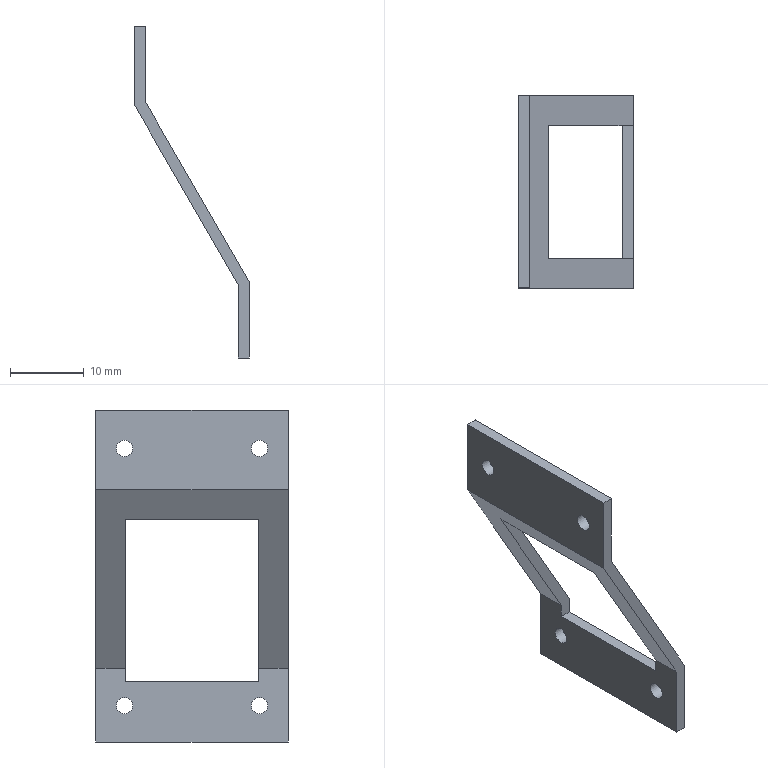Component | NX | PARTITION_PLATE | 1 solid | 18 faces | volume 1195 mm3 | plane 14 | cylinder 4 | commonest cylinder face diameters 2.2 x4